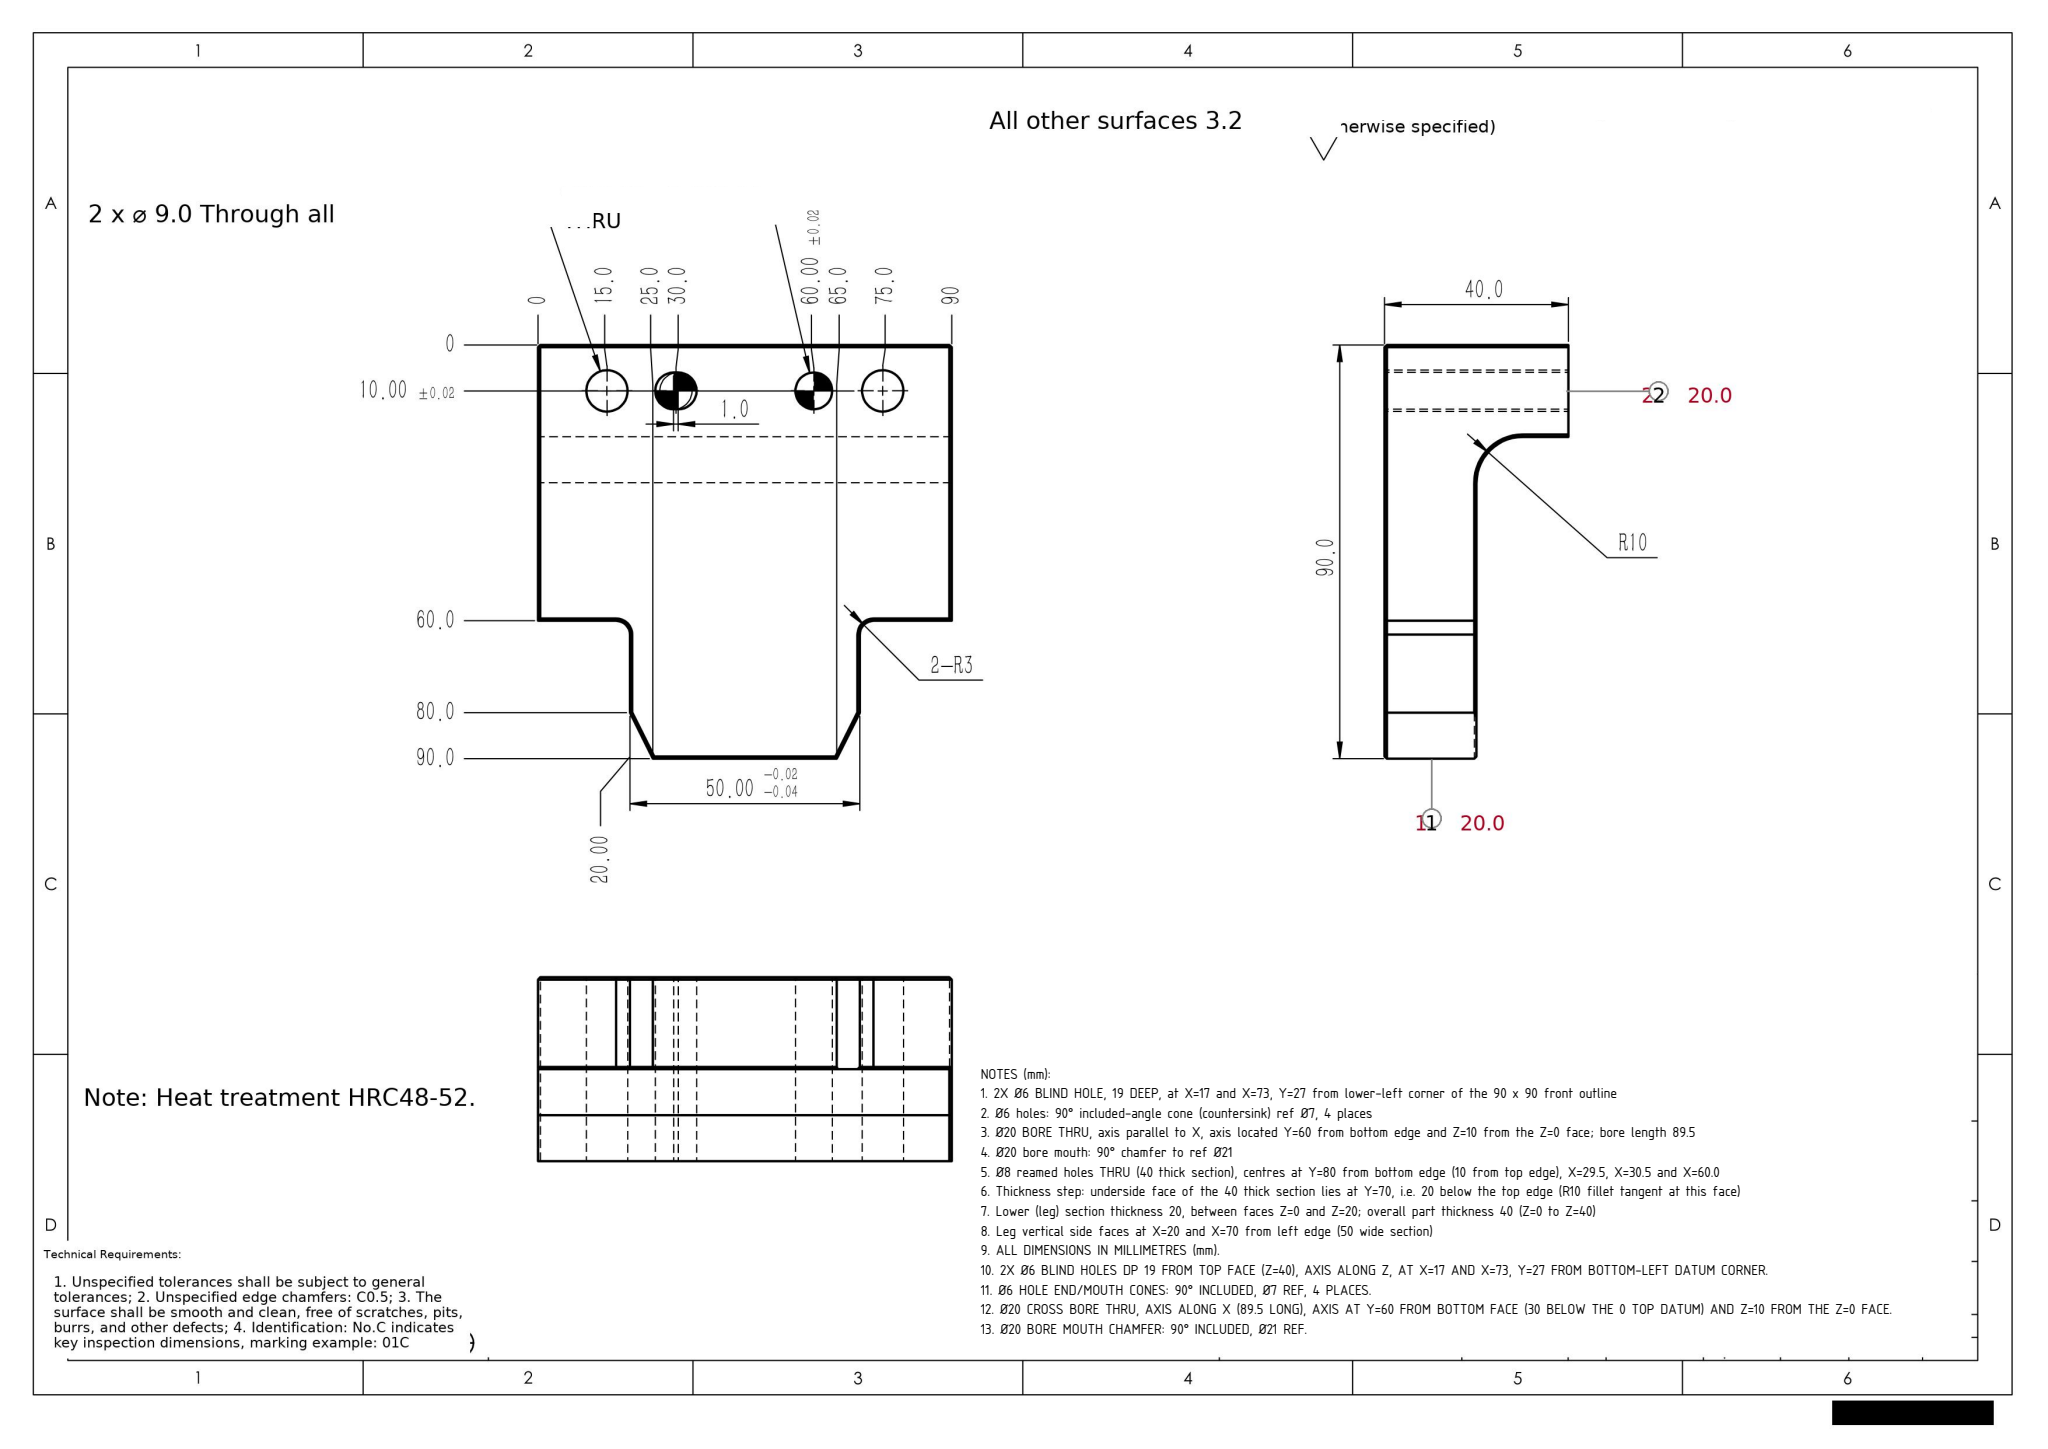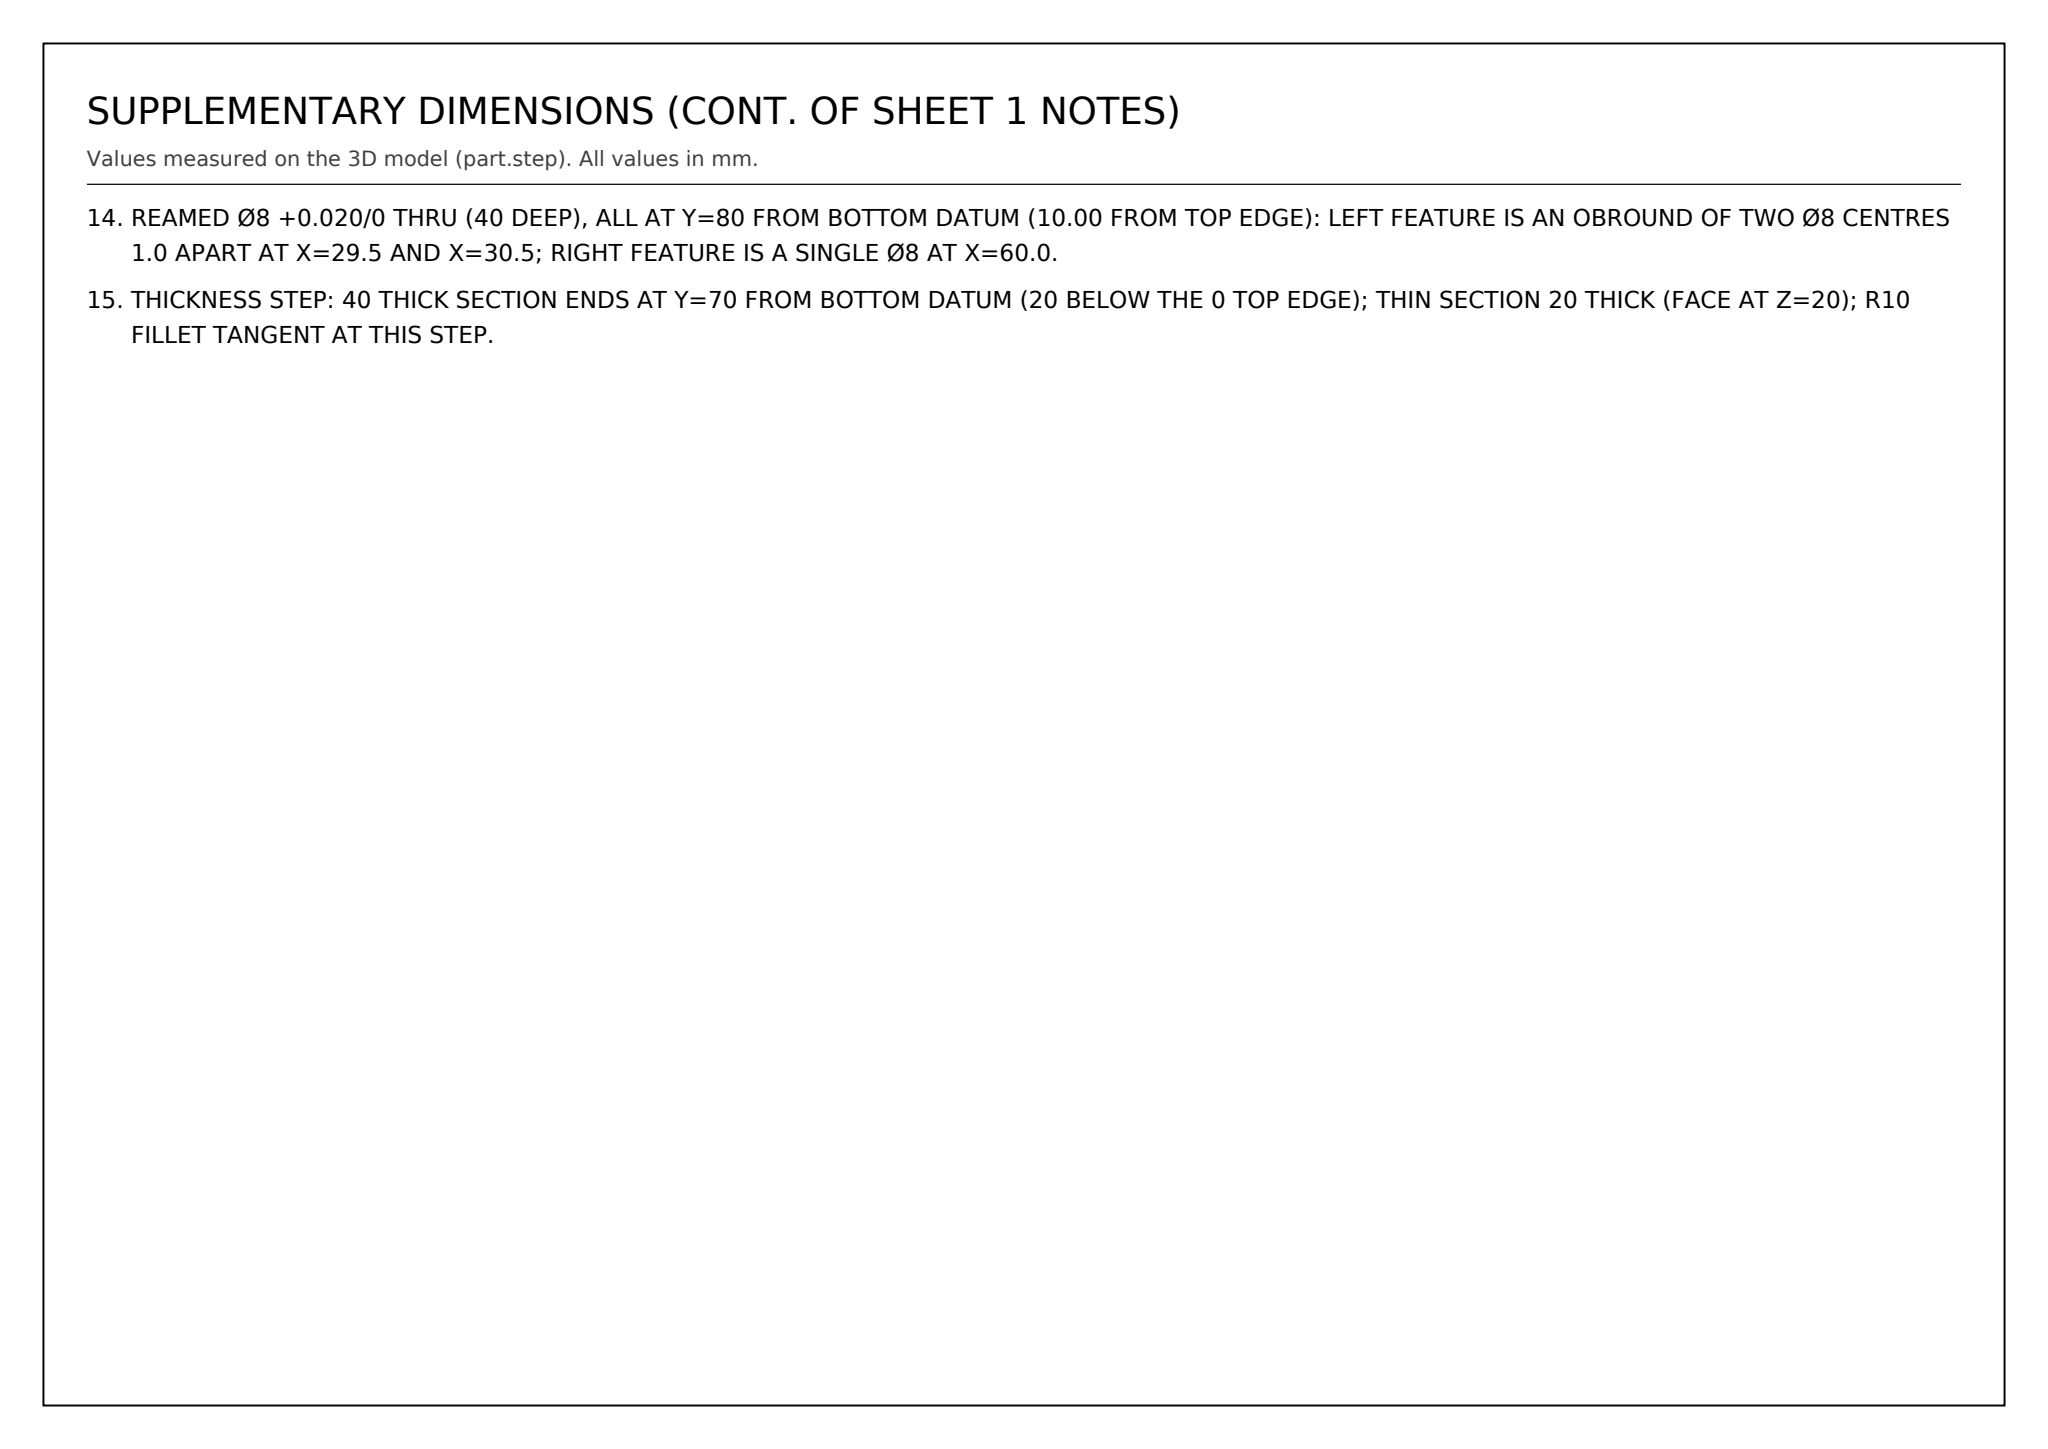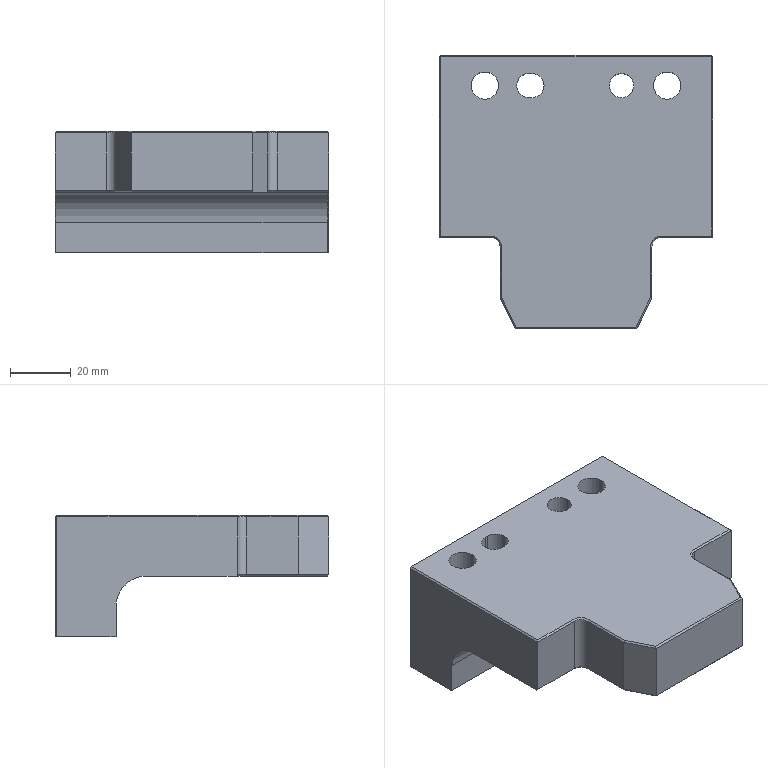Part | SolidWorks | mm | 1 solid | 55 faces | box 90 x 90 x 40 mm | volume 165501 mm3 | plane 38 | cylinder 12 | cone 5 | commonest cylinder face diameters 8 x5 9 x4 6 x2 20 x1
Drawing notes:
2X Ø6 BLIND HOLE, 19 DEEP, at X=17 and X=73, Y=27 from lower-left corner of the 90 x 90 front outline | from the solid: cylinders: [6.0,'z',[17.0,27.0],19.0] and [6.0,'z',[73.0,27.0],19.0]
Ø6 holes: 90° included-angle cone (countersink) ref Ø7, 4 places | from the solid: cones[included_angle,ref_dia]: [90.0, 7.0, 4]
Ø20 BORE THRU, axis parallel to X, axis located Y=60 from bottom edge and Z=10 from the Z=0 face; bore length 89.5 | from the solid: cylinders: [20.0,'x',[null,60.0,10.0],89.5]
Ø20 bore mouth: 90° chamfer to ref Ø21 | from the solid: cones[included_angle,ref_dia]: [90.0, 21.0, 1]
Ø8 reamed holes THRU (40 thick section), centres at Y=80 from bottom edge (10 from top edge), X=29.5, X=30.5 and X=60.0 | from the solid: cylinders: [8.0,'z',[29.5,80.0],40.0], [8.0,'z',[30.5,80.0],40.0], [8.0,'z',[60.0,80.0],40.0]
Thickness step: underside face of the 40 thick section lies at Y=70, i.e. 20 below the top edge (R10 fillet tangent at this face) | from the solid: axis_planes: ['y',70.0] with ['z',20.0] and ['z',40.0]
Lower (leg) section thickness 20, between faces Z=0 and Z=20; overall part thickness 40 (Z=0 to Z=40) | from the solid: axis_planes: ['z',0.0], ['z',20.0], ['z',40.0]; bbox_xyz Z=40
Leg vertical side faces at X=20 and X=70 from left edge (50 wide section) | from the solid: axis_planes: ['x',20.0], ['x',70.0]
ALL DIMENSIONS IN MILLIMETRES (mm). | from the solid: STEP model units mm; bbox_xyz 90.0 x 90.0 x 40.0
2X Ø6 BLIND HOLES DP 19 FROM TOP FACE (Z=40), AXIS ALONG Z, AT X=17 AND X=73, Y=27 FROM BOTTOM-LEFT DATUM CORNER. | from the solid: cylinders [6.0,'z',[17.0,27.0],19.0] and [6.0,'z',[73.0,27.0],19.0]
Ø6 HOLE END/MOUTH CONES: 90° INCLUDED, Ø7 REF, 4 PLACES. | from the solid: cones [90.0, 7.0, 4]
Ø20 CROSS BORE THRU, AXIS ALONG X (89.5 LONG), AXIS AT Y=60 FROM BOTTOM FACE (30 BELOW THE 0 TOP DATUM) AND Z=10 FROM THE Z=0 FACE. | from the solid: cylinders [20.0,'x',[y=60.0,z=10.0],89.5]
Ø20 BORE MOUTH CHAMFER: 90° INCLUDED, Ø21 REF. | from the solid: cones [90.0, 21.0, 1]
REAMED Ø8 +0.020/0 THRU (40 DEEP), ALL AT Y=80 FROM BOTTOM DATUM (10.00 FROM TOP EDGE): LEFT FEATURE IS AN OBROUND OF TWO Ø8 CENTRES 1.0 APART AT X=29.5 AND X=30.5; RIGHT FEATURE IS A SINGLE Ø8 AT X=60.0. | from the solid: cylinders 8.0 'z' at [29.5,80.0], [30.5,80.0], [60.0,80.0], length 40.0
THICKNESS STEP: 40 THICK SECTION ENDS AT Y=70 FROM BOTTOM DATUM (20 BELOW THE 0 TOP EDGE); THIN SECTION 20 THICK (FACE AT Z=20); R10 FILLET TANGENT AT THIS STEP. | from the solid: axis_planes y=70.0, z=20.0, z=40.0 (bbox Z 40.0)
build123d program:
from build123d import *

# Parameters (mm, degrees)
SKETCH1_W            = 90
SKETCH1_H            = 90
BOSS_EXTRUDE1_DEPTH  = 10
SKETCH10_W           = 90
SKETCH10_H           = 20
BOSS_EXTRUDE2_DEPTH  = 20
M8_CLEARANCE_HOLE1_D = 9
SKETCH4_R            = 4
CUT_EXTRUDE1_DEPTH   = 76.166
SKETCH5_W            = 20
SKETCH5_H            = 30
CUT_EXTRUDE2_DEPTH   = 76.166
CUT_EXTRUDE3_DEPTH   = 76.166
FILLET1_R            = 3
FILLET2_R            = 10
CHAMFER1_SIZE        = 0.5


with BuildPart() as part:
    # Sketch1 → Boss-Extrude1 (new, symmetric)
    with BuildSketch(Plane.XY):
        Rectangle(SKETCH1_W, SKETCH1_H)
    extrude(amount=BOSS_EXTRUDE1_DEPTH, both=True)

    # Sketch10 → Boss-Extrude2 (add)
    with BuildSketch(Plane(origin=(0, 0, -10), x_dir=(-1, 0, 0), z_dir=(0, 0, -1))):
        with Locations((0, 35)):
            Rectangle(SKETCH10_W, SKETCH10_H)
    extrude(amount=BOSS_EXTRUDE2_DEPTH)

    # M8 Clearance Hole1 (through all)
    with Locations(Plane.XY.offset(10)):
        with Locations((30, 35), (-30, 35)):
            Hole(M8_CLEARANCE_HOLE1_D / 2)

    # Sketch4 → Cut-Extrude1 (cut, through all)
    with BuildSketch(Plane.XY.offset(10)):
        with Locations((15, 35)):
            Circle(SKETCH4_R)
        with BuildLine():
            Line((-14.5, 31), (-15.5, 31))
            ThreePointArc((-15.5, 31), (-19.5, 35), (-15.5, 39))
            Line((-15.5, 39), (-14.5, 39))
            ThreePointArc((-14.5, 39), (-10.5, 35), (-14.5, 31))
        make_face()
    extrude(amount=-CUT_EXTRUDE1_DEPTH, mode=Mode.SUBTRACT)

    # Sketch5 → Cut-Extrude2 (cut, through all)
    with BuildSketch(Plane.XY.offset(10)):
        with Locations((35, -30)):
            Rectangle(SKETCH5_W, SKETCH5_H)
        with Locations((-35, -30)):
            Rectangle(SKETCH5_W, SKETCH5_H)
    extrude(amount=-CUT_EXTRUDE2_DEPTH, mode=Mode.SUBTRACT)

    # Sketch6 → Cut-Extrude3 (cut, through all)
    with BuildSketch(Plane.XY.offset(10)):
        Polygon((25, -45), (25, -35), (20, -45), align=None)
        Polygon((-20, -45), (-25, -45), (-25, -35), align=None)
    extrude(amount=-CUT_EXTRUDE3_DEPTH, mode=Mode.SUBTRACT)

    # Fillet1
    fillet1_edges = [part.edges().sort_by_distance(p)[0] for p in [
        (25, -15, 0),
        (-25, -15, 0),
    ]]
    fillet(fillet1_edges, radius=FILLET1_R)

    # Fillet2
    fillet2_edges = [part.edges().sort_by_distance(p)[0] for p in [
        (0, 25, -10),
    ]]
    fillet(fillet2_edges, radius=FILLET2_R)

    # Chamfer1
    chamfer1_edges = [part.edges().sort_by_distance(p)[0] for p in [
        (-45, 15, 10),
        (-25, -26.5, 10),
        (0, -45, -10),
        (0, -45, 10),
        (-22.5, -40, -10),
        (-22.5, -40, 10),
        (25, -26.5, 10),
        (36.5, -15, -10),
        (-36.5, -15, 10),
        (-25, -26.5, -10),
        (25.879, -15.879, 10),
        (25.879, -15.879, -10),
        (-25.879, -15.879, 10),
        (-25.879, -15.879, -10),
        (45, 22.071, -12.929),
        (45, 25, -25),
        (45, 0, -10),
        (45, 15, 10),
        (36.5, -15, 10),
        (0, 45, 10),
        (-36.5, -15, -10),
        (-45, 45, -10),
        (45, 45, -10),
        (25, -26.5, -10),
        (22.5, -40, 10),
    ]]
    chamfer(chamfer1_edges, length=CHAMFER1_SIZE)


solid = part.part